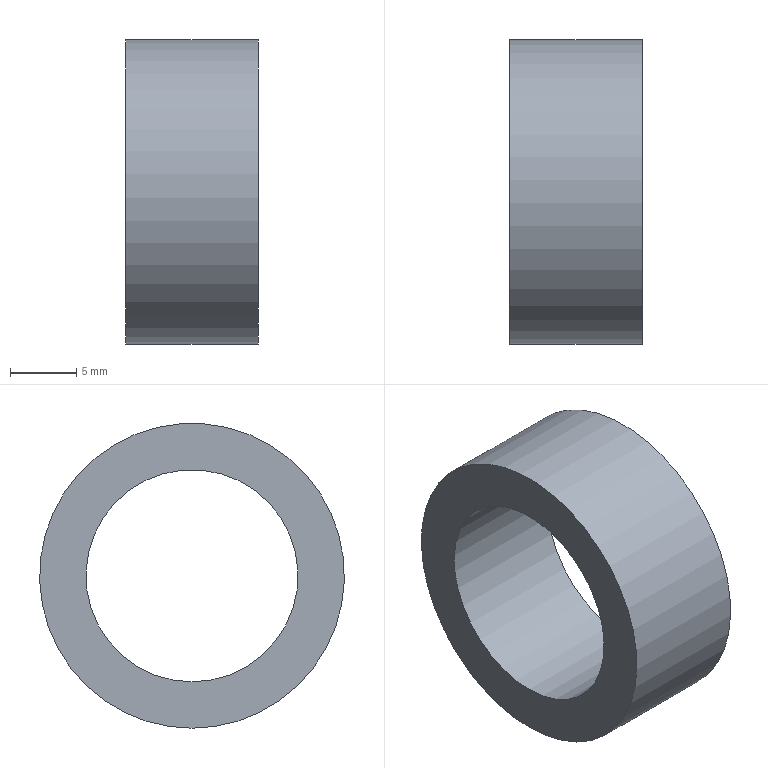Component | NX | SPACER_2 | 1 solid | 4 faces | box 10 x 23 x 23 mm | volume 2144 mm3 | cylinder 2 | plane 2 | commonest cylinder face diameters 23 x1 16 x1
STEP:
#1=CARTESIAN_POINT('',(0.,0.,0.));
#2=DIRECTION('',(0.,0.,1.));
#3=DIRECTION('',(1.,0.,0.));
#4=AXIS2_PLACEMENT_3D('',#1,#2,#3);
#5=CARTESIAN_POINT('',(-33.,-60.,-1.5));
#6=VERTEX_POINT('',#5);
#7=CARTESIAN_POINT('',(-33.,-60.,10.));
#8=DIRECTION('',(1.,0.,0.));
#9=DIRECTION('',(0.,0.,-1.));
#10=AXIS2_PLACEMENT_3D('',#7,#8,#9);
#11=CIRCLE('',#10,11.5);
#12=CARTESIAN_POINT('',(-33.,-60.,10.));
#13=DIRECTION('',(-1.,0.,0.));
#14=DIRECTION('',(0.,0.,1.));
#15=AXIS2_PLACEMENT_3D('',#12,#13,#14);
#16=CYLINDRICAL_SURFACE('',#15,11.5);
#17=CARTESIAN_POINT('',(9.425,0.));
#18=DIRECTION('',(-1.,0.));
#19=VECTOR('',#18,1.);
#20=LINE('',#17,#19);
#21=(GEOMETRIC_REPRESENTATION_CONTEXT(2)PARAMETRIC_REPRESENTATION_CONTEXT()REPRESENTATION_CONTEXT('',''));
#22=DEFINITIONAL_REPRESENTATION('',(#20),#21);
#23=PCURVE('',#16,#22);
#24=CARTESIAN_POINT('',(-33.,-60.,10.));
#25=DIRECTION('',(1.,0.,0.));
#26=DIRECTION('',(0.,0.,-1.));
#27=AXIS2_PLACEMENT_3D('',#24,#25,#26);
#28=PLANE('',#27);
#29=CARTESIAN_POINT('',(0.,0.));
#30=DIRECTION('',(1.,0.));
#31=AXIS2_PLACEMENT_2D('',#29,#30);
#32=CIRCLE('',#31,11.5);
#33=(GEOMETRIC_REPRESENTATION_CONTEXT(2)PARAMETRIC_REPRESENTATION_CONTEXT()REPRESENTATION_CONTEXT('',''));
#34=DEFINITIONAL_REPRESENTATION('',(#32),#33);
#35=PCURVE('',#28,#34);
#36=SURFACE_CURVE('',#11,(#23,#35),.PCURVE_S1.);
#37=EDGE_CURVE('',#6,#6,#36,.T.);
#38=ORIENTED_EDGE('',*,*,#37,.F.);
#39=CARTESIAN_POINT('',(-43.,-60.,-1.5));
#40=VERTEX_POINT('',#39);
#41=CARTESIAN_POINT('',(-33.,-60.,-1.5));
#42=CARTESIAN_POINT('',(-43.,-60.,-1.5));
#43=B_SPLINE_CURVE_WITH_KNOTS('',1,(#41,#42),.UNSPECIFIED.,.F.,.F.,(2,2),(0.,10.),.PIECEWISE_BEZIER_KNOTS.);
#44=CARTESIAN_POINT('',(9.425,0.));
#45=DIRECTION('',(0.,1.));
#46=VECTOR('',#45,1.);
#47=LINE('',#44,#46);
#48=(GEOMETRIC_REPRESENTATION_CONTEXT(2)PARAMETRIC_REPRESENTATION_CONTEXT()REPRESENTATION_CONTEXT('',''));
#49=DEFINITIONAL_REPRESENTATION('',(#47),#48);
#50=PCURVE('',#16,#49);
#51=CARTESIAN_POINT('',(3.142,0.));
#52=DIRECTION('',(0.,1.));
#53=VECTOR('',#52,1.);
#54=LINE('',#51,#53);
#55=(GEOMETRIC_REPRESENTATION_CONTEXT(2)PARAMETRIC_REPRESENTATION_CONTEXT()REPRESENTATION_CONTEXT('',''));
#56=DEFINITIONAL_REPRESENTATION('',(#54),#55);
#57=PCURVE('',#16,#56);
#58=SEAM_CURVE('',#43,(#50,#57),.PCURVE_S1.);
#59=EDGE_CURVE('',#6,#40,#58,.T.);
#60=ORIENTED_EDGE('',*,*,#59,.T.);
#61=CARTESIAN_POINT('',(-43.,-60.,10.));
#62=DIRECTION('',(1.,0.,0.));
#63=DIRECTION('',(0.,0.,-1.));
#64=AXIS2_PLACEMENT_3D('',#61,#62,#63);
#65=CIRCLE('',#64,11.5);
#66=CARTESIAN_POINT('',(9.425,10.));
#67=DIRECTION('',(-1.,0.));
#68=VECTOR('',#67,1.);
#69=LINE('',#66,#68);
#70=(GEOMETRIC_REPRESENTATION_CONTEXT(2)PARAMETRIC_REPRESENTATION_CONTEXT()REPRESENTATION_CONTEXT('',''));
#71=DEFINITIONAL_REPRESENTATION('',(#69),#70);
#72=PCURVE('',#16,#71);
#73=CARTESIAN_POINT('',(-43.,-60.,10.));
#74=DIRECTION('',(1.,0.,0.));
#75=DIRECTION('',(0.,0.,-1.));
#76=AXIS2_PLACEMENT_3D('',#73,#74,#75);
#77=PLANE('',#76);
#78=CARTESIAN_POINT('',(0.,0.));
#79=DIRECTION('',(1.,0.));
#80=AXIS2_PLACEMENT_2D('',#78,#79);
#81=CIRCLE('',#80,11.5);
#82=(GEOMETRIC_REPRESENTATION_CONTEXT(2)PARAMETRIC_REPRESENTATION_CONTEXT()REPRESENTATION_CONTEXT('',''));
#83=DEFINITIONAL_REPRESENTATION('',(#81),#82);
#84=PCURVE('',#77,#83);
#85=SURFACE_CURVE('',#65,(#72,#84),.PCURVE_S1.);
#86=EDGE_CURVE('',#40,#40,#85,.T.);
#87=ORIENTED_EDGE('',*,*,#86,.T.);
#88=ORIENTED_EDGE('',*,*,#59,.F.);
#89=EDGE_LOOP('',(#38,#60,#87,#88));
#90=FACE_BOUND('',#89,.T.);
#91=ADVANCED_FACE('',(#90),#16,.T.);
#92=CARTESIAN_POINT('',(-33.,-60.,2.));
#93=VERTEX_POINT('',#92);
#94=CARTESIAN_POINT('',(-33.,-60.,10.));
#95=DIRECTION('',(1.,0.,0.));
#96=DIRECTION('',(0.,0.,-1.));
#97=AXIS2_PLACEMENT_3D('',#94,#95,#96);
#98=CIRCLE('',#97,8.);
#99=CARTESIAN_POINT('',(-33.,-60.,10.));
#100=DIRECTION('',(-1.,0.,0.));
#101=DIRECTION('',(0.,0.,1.));
#102=AXIS2_PLACEMENT_3D('',#99,#100,#101);
#103=CYLINDRICAL_SURFACE('',#102,8.);
#104=CARTESIAN_POINT('',(9.425,0.));
#105=DIRECTION('',(-1.,0.));
#106=VECTOR('',#105,1.);
#107=LINE('',#104,#106);
#108=(GEOMETRIC_REPRESENTATION_CONTEXT(2)PARAMETRIC_REPRESENTATION_CONTEXT()REPRESENTATION_CONTEXT('',''));
#109=DEFINITIONAL_REPRESENTATION('',(#107),#108);
#110=PCURVE('',#103,#109);
#111=CARTESIAN_POINT('',(0.,0.));
#112=DIRECTION('',(1.,0.));
#113=AXIS2_PLACEMENT_2D('',#111,#112);
#114=CIRCLE('',#113,8.);
#115=(GEOMETRIC_REPRESENTATION_CONTEXT(2)PARAMETRIC_REPRESENTATION_CONTEXT()REPRESENTATION_CONTEXT('',''));
#116=DEFINITIONAL_REPRESENTATION('',(#114),#115);
#117=PCURVE('',#28,#116);
#118=SURFACE_CURVE('',#98,(#110,#117),.PCURVE_S1.);
#119=EDGE_CURVE('',#93,#93,#118,.T.);
#120=ORIENTED_EDGE('',*,*,#119,.F.);
#121=CARTESIAN_POINT('',(-43.,-60.,2.));
#122=VERTEX_POINT('',#121);
#123=CARTESIAN_POINT('',(-33.,-60.,2.));
#124=CARTESIAN_POINT('',(-43.,-60.,2.));
#125=B_SPLINE_CURVE_WITH_KNOTS('',1,(#123,#124),.UNSPECIFIED.,.F.,.F.,(2,2),(0.,10.),.PIECEWISE_BEZIER_KNOTS.);
#126=CARTESIAN_POINT('',(9.425,0.));
#127=DIRECTION('',(0.,1.));
#128=VECTOR('',#127,1.);
#129=LINE('',#126,#128);
#130=(GEOMETRIC_REPRESENTATION_CONTEXT(2)PARAMETRIC_REPRESENTATION_CONTEXT()REPRESENTATION_CONTEXT('',''));
#131=DEFINITIONAL_REPRESENTATION('',(#129),#130);
#132=PCURVE('',#103,#131);
#133=CARTESIAN_POINT('',(3.142,0.));
#134=DIRECTION('',(0.,1.));
#135=VECTOR('',#134,1.);
#136=LINE('',#133,#135);
#137=(GEOMETRIC_REPRESENTATION_CONTEXT(2)PARAMETRIC_REPRESENTATION_CONTEXT()REPRESENTATION_CONTEXT('',''));
#138=DEFINITIONAL_REPRESENTATION('',(#136),#137);
#139=PCURVE('',#103,#138);
#140=SEAM_CURVE('',#125,(#132,#139),.PCURVE_S1.);
#141=EDGE_CURVE('',#93,#122,#140,.T.);
#142=ORIENTED_EDGE('',*,*,#141,.T.);
#143=CARTESIAN_POINT('',(-43.,-60.,10.));
#144=DIRECTION('',(1.,0.,0.));
#145=DIRECTION('',(0.,0.,-1.));
#146=AXIS2_PLACEMENT_3D('',#143,#144,#145);
#147=CIRCLE('',#146,8.);
#148=CARTESIAN_POINT('',(9.425,10.));
#149=DIRECTION('',(-1.,0.));
#150=VECTOR('',#149,1.);
#151=LINE('',#148,#150);
#152=(GEOMETRIC_REPRESENTATION_CONTEXT(2)PARAMETRIC_REPRESENTATION_CONTEXT()REPRESENTATION_CONTEXT('',''));
#153=DEFINITIONAL_REPRESENTATION('',(#151),#152);
#154=PCURVE('',#103,#153);
#155=CARTESIAN_POINT('',(0.,0.));
#156=DIRECTION('',(1.,0.));
#157=AXIS2_PLACEMENT_2D('',#155,#156);
#158=CIRCLE('',#157,8.);
#159=(GEOMETRIC_REPRESENTATION_CONTEXT(2)PARAMETRIC_REPRESENTATION_CONTEXT()REPRESENTATION_CONTEXT('',''));
#160=DEFINITIONAL_REPRESENTATION('',(#158),#159);
#161=PCURVE('',#77,#160);
#162=SURFACE_CURVE('',#147,(#154,#161),.PCURVE_S1.);
#163=EDGE_CURVE('',#122,#122,#162,.T.);
#164=ORIENTED_EDGE('',*,*,#163,.T.);
#165=ORIENTED_EDGE('',*,*,#141,.F.);
#166=EDGE_LOOP('',(#120,#142,#164,#165));
#167=FACE_BOUND('',#166,.F.);
#168=ADVANCED_FACE('',(#167),#103,.F.);
#169=ORIENTED_EDGE('',*,*,#37,.T.);
#170=EDGE_LOOP('',(#169));
#171=FACE_BOUND('',#170,.T.);
#172=ORIENTED_EDGE('',*,*,#119,.F.);
#173=EDGE_LOOP('',(#172));
#174=FACE_BOUND('',#173,.T.);
#175=ADVANCED_FACE('',(#171,#174),#28,.T.);
#176=ORIENTED_EDGE('',*,*,#86,.F.);
#177=EDGE_LOOP('',(#176));
#178=FACE_BOUND('',#177,.T.);
#179=ORIENTED_EDGE('',*,*,#163,.T.);
#180=EDGE_LOOP('',(#179));
#181=FACE_BOUND('',#180,.T.);
#182=ADVANCED_FACE('',(#178,#181),#77,.F.);
#183=CLOSED_SHELL('',(#91,#168,#175,#182));
#184=MANIFOLD_SOLID_BREP('',#183);
#185=(LENGTH_UNIT()NAMED_UNIT(*)SI_UNIT(.MILLI.,.METRE.));
#186=UNCERTAINTY_MEASURE_WITH_UNIT(LENGTH_MEASURE(0.00001),#185,'','');
#187=(NAMED_UNIT(*)PLANE_ANGLE_UNIT()SI_UNIT($,.RADIAN.));
#188=(NAMED_UNIT(*)SI_UNIT($,.STERADIAN.)SOLID_ANGLE_UNIT());
#189=(GEOMETRIC_REPRESENTATION_CONTEXT(3)GLOBAL_UNCERTAINTY_ASSIGNED_CONTEXT((#186))GLOBAL_UNIT_ASSIGNED_CONTEXT((#185,#187,#188))REPRESENTATION_CONTEXT('',''));
#190=ADVANCED_BREP_SHAPE_REPRESENTATION('',(#4,#184),#189);